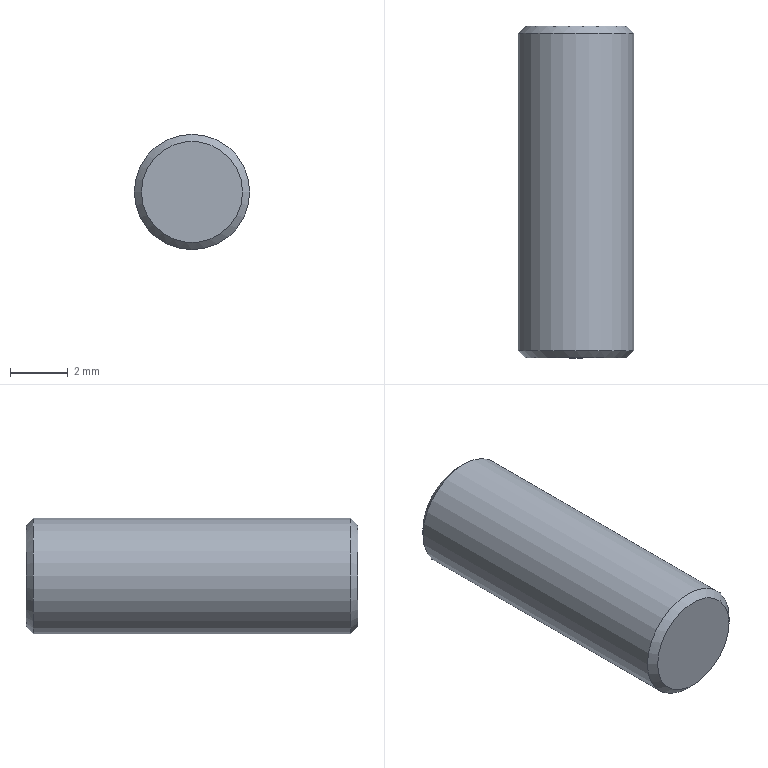Component | NX | CONNECTING_ROD_JOINT_1_CONNECTING_SHAFT_3 | 1 solid | 5 faces | box 4 x 11.5 x 4 mm | volume 144 mm3 | plane 2 | cone 2 | cylinder 1 | commonest cylinder face diameters 4 x1
STEP:
#1=CARTESIAN_POINT('',(0.,0.,0.));
#2=DIRECTION('',(0.,0.,1.));
#3=DIRECTION('',(1.,0.,0.));
#4=AXIS2_PLACEMENT_3D('',#1,#2,#3);
#5=CARTESIAN_POINT('',(8.951,-42.5,41.));
#6=VERTEX_POINT('',#5);
#7=CARTESIAN_POINT('',(7.201,-42.5,41.));
#8=DIRECTION('',(0.,-1.,0.));
#9=DIRECTION('',(1.,0.,0.));
#10=AXIS2_PLACEMENT_3D('',#7,#8,#9);
#11=CIRCLE('',#10,1.75);
#12=CARTESIAN_POINT('',(7.201,-42.5,41.));
#13=DIRECTION('',(0.,-1.,0.));
#14=DIRECTION('',(1.,0.,0.));
#15=AXIS2_PLACEMENT_3D('',#12,#13,#14);
#16=PLANE('',#15);
#17=CARTESIAN_POINT('',(0.,0.));
#18=DIRECTION('',(1.,0.));
#19=AXIS2_PLACEMENT_2D('',#17,#18);
#20=CIRCLE('',#19,1.75);
#21=(GEOMETRIC_REPRESENTATION_CONTEXT(2)PARAMETRIC_REPRESENTATION_CONTEXT()REPRESENTATION_CONTEXT('',''));
#22=DEFINITIONAL_REPRESENTATION('',(#20),#21);
#23=PCURVE('',#16,#22);
#24=CARTESIAN_POINT('',(7.201,-42.25,41.));
#25=DIRECTION('',(0.,1.,0.));
#26=DIRECTION('',(-1.,0.,0.));
#27=AXIS2_PLACEMENT_3D('',#24,#25,#26);
#28=CONICAL_SURFACE('',#27,2.,0.7854);
#29=CARTESIAN_POINT('',(9.425,-0.25));
#30=DIRECTION('',(-1.,0.));
#31=VECTOR('',#30,1.);
#32=LINE('',#29,#31);
#33=(GEOMETRIC_REPRESENTATION_CONTEXT(2)PARAMETRIC_REPRESENTATION_CONTEXT()REPRESENTATION_CONTEXT('',''));
#34=DEFINITIONAL_REPRESENTATION('',(#32),#33);
#35=PCURVE('',#28,#34);
#36=SURFACE_CURVE('',#11,(#23,#35),.PCURVE_S1.);
#37=EDGE_CURVE('',#6,#6,#36,.T.);
#38=ORIENTED_EDGE('',*,*,#37,.T.);
#39=EDGE_LOOP('',(#38));
#40=FACE_BOUND('',#39,.T.);
#41=ADVANCED_FACE('',(#40),#16,.T.);
#42=CARTESIAN_POINT('',(5.451,-31.,41.));
#43=VERTEX_POINT('',#42);
#44=CARTESIAN_POINT('',(7.201,-31.,41.));
#45=DIRECTION('',(0.,1.,0.));
#46=DIRECTION('',(-1.,0.,0.));
#47=AXIS2_PLACEMENT_3D('',#44,#45,#46);
#48=CIRCLE('',#47,1.75);
#49=CARTESIAN_POINT('',(7.201,-31.,41.));
#50=DIRECTION('',(0.,1.,0.));
#51=DIRECTION('',(-1.,0.,0.));
#52=AXIS2_PLACEMENT_3D('',#49,#50,#51);
#53=PLANE('',#52);
#54=CARTESIAN_POINT('',(0.,0.));
#55=DIRECTION('',(1.,0.));
#56=AXIS2_PLACEMENT_2D('',#54,#55);
#57=CIRCLE('',#56,1.75);
#58=(GEOMETRIC_REPRESENTATION_CONTEXT(2)PARAMETRIC_REPRESENTATION_CONTEXT()REPRESENTATION_CONTEXT('',''));
#59=DEFINITIONAL_REPRESENTATION('',(#57),#58);
#60=PCURVE('',#53,#59);
#61=CARTESIAN_POINT('',(7.201,-31.25,41.));
#62=DIRECTION('',(0.,-1.,0.));
#63=DIRECTION('',(1.,0.,0.));
#64=AXIS2_PLACEMENT_3D('',#61,#62,#63);
#65=CONICAL_SURFACE('',#64,2.,0.7854);
#66=CARTESIAN_POINT('',(9.425,-0.25));
#67=DIRECTION('',(-1.,0.));
#68=VECTOR('',#67,1.);
#69=LINE('',#66,#68);
#70=(GEOMETRIC_REPRESENTATION_CONTEXT(2)PARAMETRIC_REPRESENTATION_CONTEXT()REPRESENTATION_CONTEXT('',''));
#71=DEFINITIONAL_REPRESENTATION('',(#69),#70);
#72=PCURVE('',#65,#71);
#73=SURFACE_CURVE('',#48,(#60,#72),.PCURVE_S1.);
#74=EDGE_CURVE('',#43,#43,#73,.T.);
#75=ORIENTED_EDGE('',*,*,#74,.T.);
#76=EDGE_LOOP('',(#75));
#77=FACE_BOUND('',#76,.T.);
#78=ADVANCED_FACE('',(#77),#53,.T.);
#79=CARTESIAN_POINT('',(5.201,-31.25,41.));
#80=VERTEX_POINT('',#79);
#81=CARTESIAN_POINT('',(9.201,-31.25,41.));
#82=VERTEX_POINT('',#81);
#83=CARTESIAN_POINT('',(7.201,-31.25,41.));
#84=DIRECTION('',(0.,-1.,0.));
#85=DIRECTION('',(-1.,0.,0.));
#86=AXIS2_PLACEMENT_3D('',#83,#84,#85);
#87=CIRCLE('',#86,2.);
#88=CARTESIAN_POINT('',(7.201,-31.,41.));
#89=DIRECTION('',(0.,-1.,0.));
#90=DIRECTION('',(1.,0.,0.));
#91=AXIS2_PLACEMENT_3D('',#88,#89,#90);
#92=CYLINDRICAL_SURFACE('',#91,2.);
#93=CARTESIAN_POINT('',(3.142,0.25));
#94=DIRECTION('',(1.,0.));
#95=VECTOR('',#94,1.);
#96=LINE('',#93,#95);
#97=(GEOMETRIC_REPRESENTATION_CONTEXT(2)PARAMETRIC_REPRESENTATION_CONTEXT()REPRESENTATION_CONTEXT('',''));
#98=DEFINITIONAL_REPRESENTATION('',(#96),#97);
#99=PCURVE('',#92,#98);
#100=CARTESIAN_POINT('',(3.142,0.));
#101=DIRECTION('',(1.,0.));
#102=VECTOR('',#101,1.);
#103=LINE('',#100,#102);
#104=(GEOMETRIC_REPRESENTATION_CONTEXT(2)PARAMETRIC_REPRESENTATION_CONTEXT()REPRESENTATION_CONTEXT('',''));
#105=DEFINITIONAL_REPRESENTATION('',(#103),#104);
#106=PCURVE('',#65,#105);
#107=SURFACE_CURVE('',#87,(#99,#106),.PCURVE_S1.);
#108=EDGE_CURVE('',#80,#82,#107,.T.);
#109=ORIENTED_EDGE('',*,*,#108,.T.);
#110=CARTESIAN_POINT('',(9.201,-42.25,41.));
#111=VERTEX_POINT('',#110);
#112=CARTESIAN_POINT('',(9.201,-31.25,41.));
#113=CARTESIAN_POINT('',(9.201,-42.25,41.));
#114=B_SPLINE_CURVE_WITH_KNOTS('',1,(#112,#113),.UNSPECIFIED.,.F.,.F.,(2,2),(0.25,11.25),.PIECEWISE_BEZIER_KNOTS.);
#115=CARTESIAN_POINT('',(6.283,0.));
#116=DIRECTION('',(0.,1.));
#117=VECTOR('',#116,1.);
#118=LINE('',#115,#117);
#119=(GEOMETRIC_REPRESENTATION_CONTEXT(2)PARAMETRIC_REPRESENTATION_CONTEXT()REPRESENTATION_CONTEXT('',''));
#120=DEFINITIONAL_REPRESENTATION('',(#118),#119);
#121=PCURVE('',#92,#120);
#122=CARTESIAN_POINT('',(0.,0.));
#123=DIRECTION('',(0.,1.));
#124=VECTOR('',#123,1.);
#125=LINE('',#122,#124);
#126=(GEOMETRIC_REPRESENTATION_CONTEXT(2)PARAMETRIC_REPRESENTATION_CONTEXT()REPRESENTATION_CONTEXT('',''));
#127=DEFINITIONAL_REPRESENTATION('',(#125),#126);
#128=PCURVE('',#92,#127);
#129=SEAM_CURVE('',#114,(#121,#128),.PCURVE_S1.);
#130=EDGE_CURVE('',#82,#111,#129,.T.);
#131=ORIENTED_EDGE('',*,*,#130,.T.);
#132=CARTESIAN_POINT('',(7.201,-42.25,41.));
#133=DIRECTION('',(0.,1.,0.));
#134=DIRECTION('',(1.,0.,0.));
#135=AXIS2_PLACEMENT_3D('',#132,#133,#134);
#136=CIRCLE('',#135,2.);
#137=CARTESIAN_POINT('',(6.283,11.25));
#138=DIRECTION('',(-1.,0.));
#139=VECTOR('',#138,1.);
#140=LINE('',#137,#139);
#141=(GEOMETRIC_REPRESENTATION_CONTEXT(2)PARAMETRIC_REPRESENTATION_CONTEXT()REPRESENTATION_CONTEXT('',''));
#142=DEFINITIONAL_REPRESENTATION('',(#140),#141);
#143=PCURVE('',#92,#142);
#144=CARTESIAN_POINT('',(3.142,0.));
#145=DIRECTION('',(1.,0.));
#146=VECTOR('',#145,1.);
#147=LINE('',#144,#146);
#148=(GEOMETRIC_REPRESENTATION_CONTEXT(2)PARAMETRIC_REPRESENTATION_CONTEXT()REPRESENTATION_CONTEXT('',''));
#149=DEFINITIONAL_REPRESENTATION('',(#147),#148);
#150=PCURVE('',#28,#149);
#151=SURFACE_CURVE('',#136,(#143,#150),.PCURVE_S1.);
#152=EDGE_CURVE('',#111,#111,#151,.T.);
#153=ORIENTED_EDGE('',*,*,#152,.T.);
#154=ORIENTED_EDGE('',*,*,#130,.F.);
#155=CARTESIAN_POINT('',(7.201,-31.25,41.));
#156=DIRECTION('',(0.,-1.,0.));
#157=DIRECTION('',(-1.,0.,0.));
#158=AXIS2_PLACEMENT_3D('',#155,#156,#157);
#159=CIRCLE('',#158,2.);
#160=CARTESIAN_POINT('',(-3.142,0.25));
#161=DIRECTION('',(1.,0.));
#162=VECTOR('',#161,1.);
#163=LINE('',#160,#162);
#164=(GEOMETRIC_REPRESENTATION_CONTEXT(2)PARAMETRIC_REPRESENTATION_CONTEXT()REPRESENTATION_CONTEXT('',''));
#165=DEFINITIONAL_REPRESENTATION('',(#163),#164);
#166=PCURVE('',#92,#165);
#167=CARTESIAN_POINT('',(3.142,0.));
#168=DIRECTION('',(1.,0.));
#169=VECTOR('',#168,1.);
#170=LINE('',#167,#169);
#171=(GEOMETRIC_REPRESENTATION_CONTEXT(2)PARAMETRIC_REPRESENTATION_CONTEXT()REPRESENTATION_CONTEXT('',''));
#172=DEFINITIONAL_REPRESENTATION('',(#170),#171);
#173=PCURVE('',#65,#172);
#174=SURFACE_CURVE('',#159,(#166,#173),.PCURVE_S1.);
#175=EDGE_CURVE('',#82,#80,#174,.T.);
#176=ORIENTED_EDGE('',*,*,#175,.T.);
#177=EDGE_LOOP('',(#109,#131,#153,#154,#176));
#178=FACE_BOUND('',#177,.T.);
#179=ADVANCED_FACE('',(#178),#92,.T.);
#180=ORIENTED_EDGE('',*,*,#74,.F.);
#181=CARTESIAN_POINT('',(5.451,-31.,41.));
#182=CARTESIAN_POINT('',(5.201,-31.25,41.));
#183=B_SPLINE_CURVE_WITH_KNOTS('',1,(#181,#182),.UNSPECIFIED.,.F.,.F.,(2,2),(-0.3536,0.),.PIECEWISE_BEZIER_KNOTS.);
#184=CARTESIAN_POINT('',(9.425,0.));
#185=DIRECTION('',(0.,1.));
#186=VECTOR('',#185,1.);
#187=LINE('',#184,#186);
#188=(GEOMETRIC_REPRESENTATION_CONTEXT(2)PARAMETRIC_REPRESENTATION_CONTEXT()REPRESENTATION_CONTEXT('',''));
#189=DEFINITIONAL_REPRESENTATION('',(#187),#188);
#190=PCURVE('',#65,#189);
#191=CARTESIAN_POINT('',(3.142,0.));
#192=DIRECTION('',(0.,1.));
#193=VECTOR('',#192,1.);
#194=LINE('',#191,#193);
#195=(GEOMETRIC_REPRESENTATION_CONTEXT(2)PARAMETRIC_REPRESENTATION_CONTEXT()REPRESENTATION_CONTEXT('',''));
#196=DEFINITIONAL_REPRESENTATION('',(#194),#195);
#197=PCURVE('',#65,#196);
#198=SEAM_CURVE('',#183,(#190,#197),.PCURVE_S1.);
#199=EDGE_CURVE('',#43,#80,#198,.T.);
#200=ORIENTED_EDGE('',*,*,#199,.T.);
#201=ORIENTED_EDGE('',*,*,#175,.F.);
#202=ORIENTED_EDGE('',*,*,#108,.F.);
#203=ORIENTED_EDGE('',*,*,#199,.F.);
#204=EDGE_LOOP('',(#180,#200,#201,#202,#203));
#205=FACE_BOUND('',#204,.T.);
#206=ADVANCED_FACE('',(#205),#65,.T.);
#207=ORIENTED_EDGE('',*,*,#37,.F.);
#208=CARTESIAN_POINT('',(8.951,-42.5,41.));
#209=CARTESIAN_POINT('',(9.201,-42.25,41.));
#210=B_SPLINE_CURVE_WITH_KNOTS('',1,(#208,#209),.UNSPECIFIED.,.F.,.F.,(2,2),(-0.3536,0.),.PIECEWISE_BEZIER_KNOTS.);
#211=CARTESIAN_POINT('',(9.425,0.));
#212=DIRECTION('',(0.,1.));
#213=VECTOR('',#212,1.);
#214=LINE('',#211,#213);
#215=(GEOMETRIC_REPRESENTATION_CONTEXT(2)PARAMETRIC_REPRESENTATION_CONTEXT()REPRESENTATION_CONTEXT('',''));
#216=DEFINITIONAL_REPRESENTATION('',(#214),#215);
#217=PCURVE('',#28,#216);
#218=CARTESIAN_POINT('',(3.142,0.));
#219=DIRECTION('',(0.,1.));
#220=VECTOR('',#219,1.);
#221=LINE('',#218,#220);
#222=(GEOMETRIC_REPRESENTATION_CONTEXT(2)PARAMETRIC_REPRESENTATION_CONTEXT()REPRESENTATION_CONTEXT('',''));
#223=DEFINITIONAL_REPRESENTATION('',(#221),#222);
#224=PCURVE('',#28,#223);
#225=SEAM_CURVE('',#210,(#217,#224),.PCURVE_S1.);
#226=EDGE_CURVE('',#6,#111,#225,.T.);
#227=ORIENTED_EDGE('',*,*,#226,.T.);
#228=ORIENTED_EDGE('',*,*,#152,.F.);
#229=ORIENTED_EDGE('',*,*,#226,.F.);
#230=EDGE_LOOP('',(#207,#227,#228,#229));
#231=FACE_BOUND('',#230,.T.);
#232=ADVANCED_FACE('',(#231),#28,.T.);
#233=CLOSED_SHELL('',(#41,#78,#179,#206,#232));
#234=MANIFOLD_SOLID_BREP('',#233);
#235=(LENGTH_UNIT()NAMED_UNIT(*)SI_UNIT(.MILLI.,.METRE.));
#236=UNCERTAINTY_MEASURE_WITH_UNIT(LENGTH_MEASURE(0.00001),#235,'','');
#237=(NAMED_UNIT(*)PLANE_ANGLE_UNIT()SI_UNIT($,.RADIAN.));
#238=(NAMED_UNIT(*)SI_UNIT($,.STERADIAN.)SOLID_ANGLE_UNIT());
#239=(GEOMETRIC_REPRESENTATION_CONTEXT(3)GLOBAL_UNCERTAINTY_ASSIGNED_CONTEXT((#236))GLOBAL_UNIT_ASSIGNED_CONTEXT((#235,#237,#238))REPRESENTATION_CONTEXT('',''));
#240=ADVANCED_BREP_SHAPE_REPRESENTATION('',(#4,#234),#239);